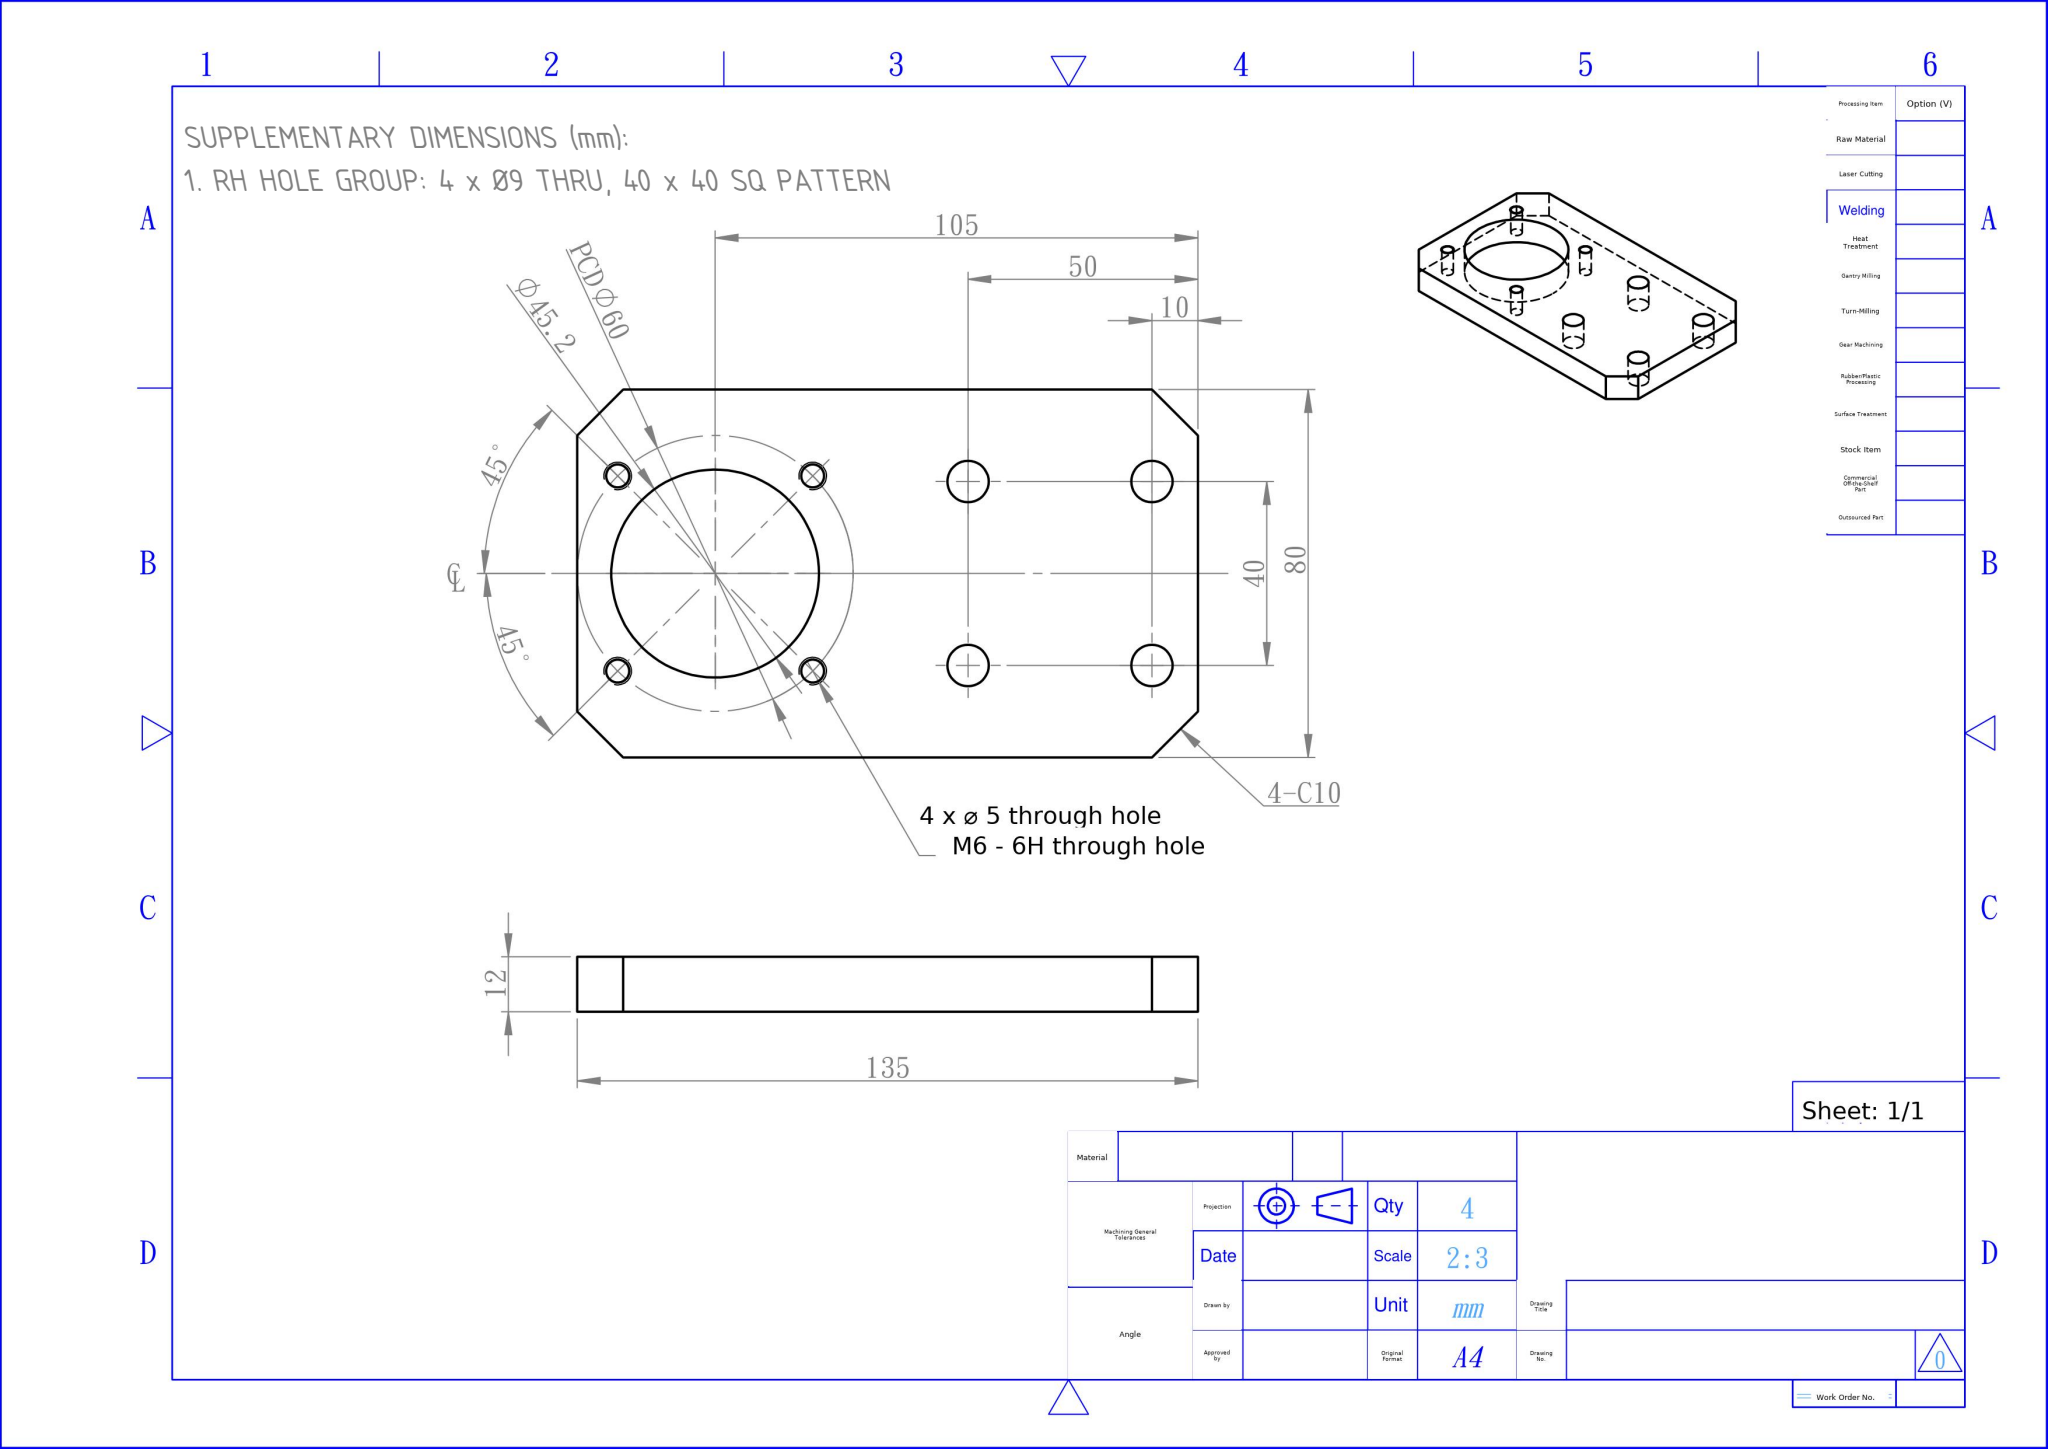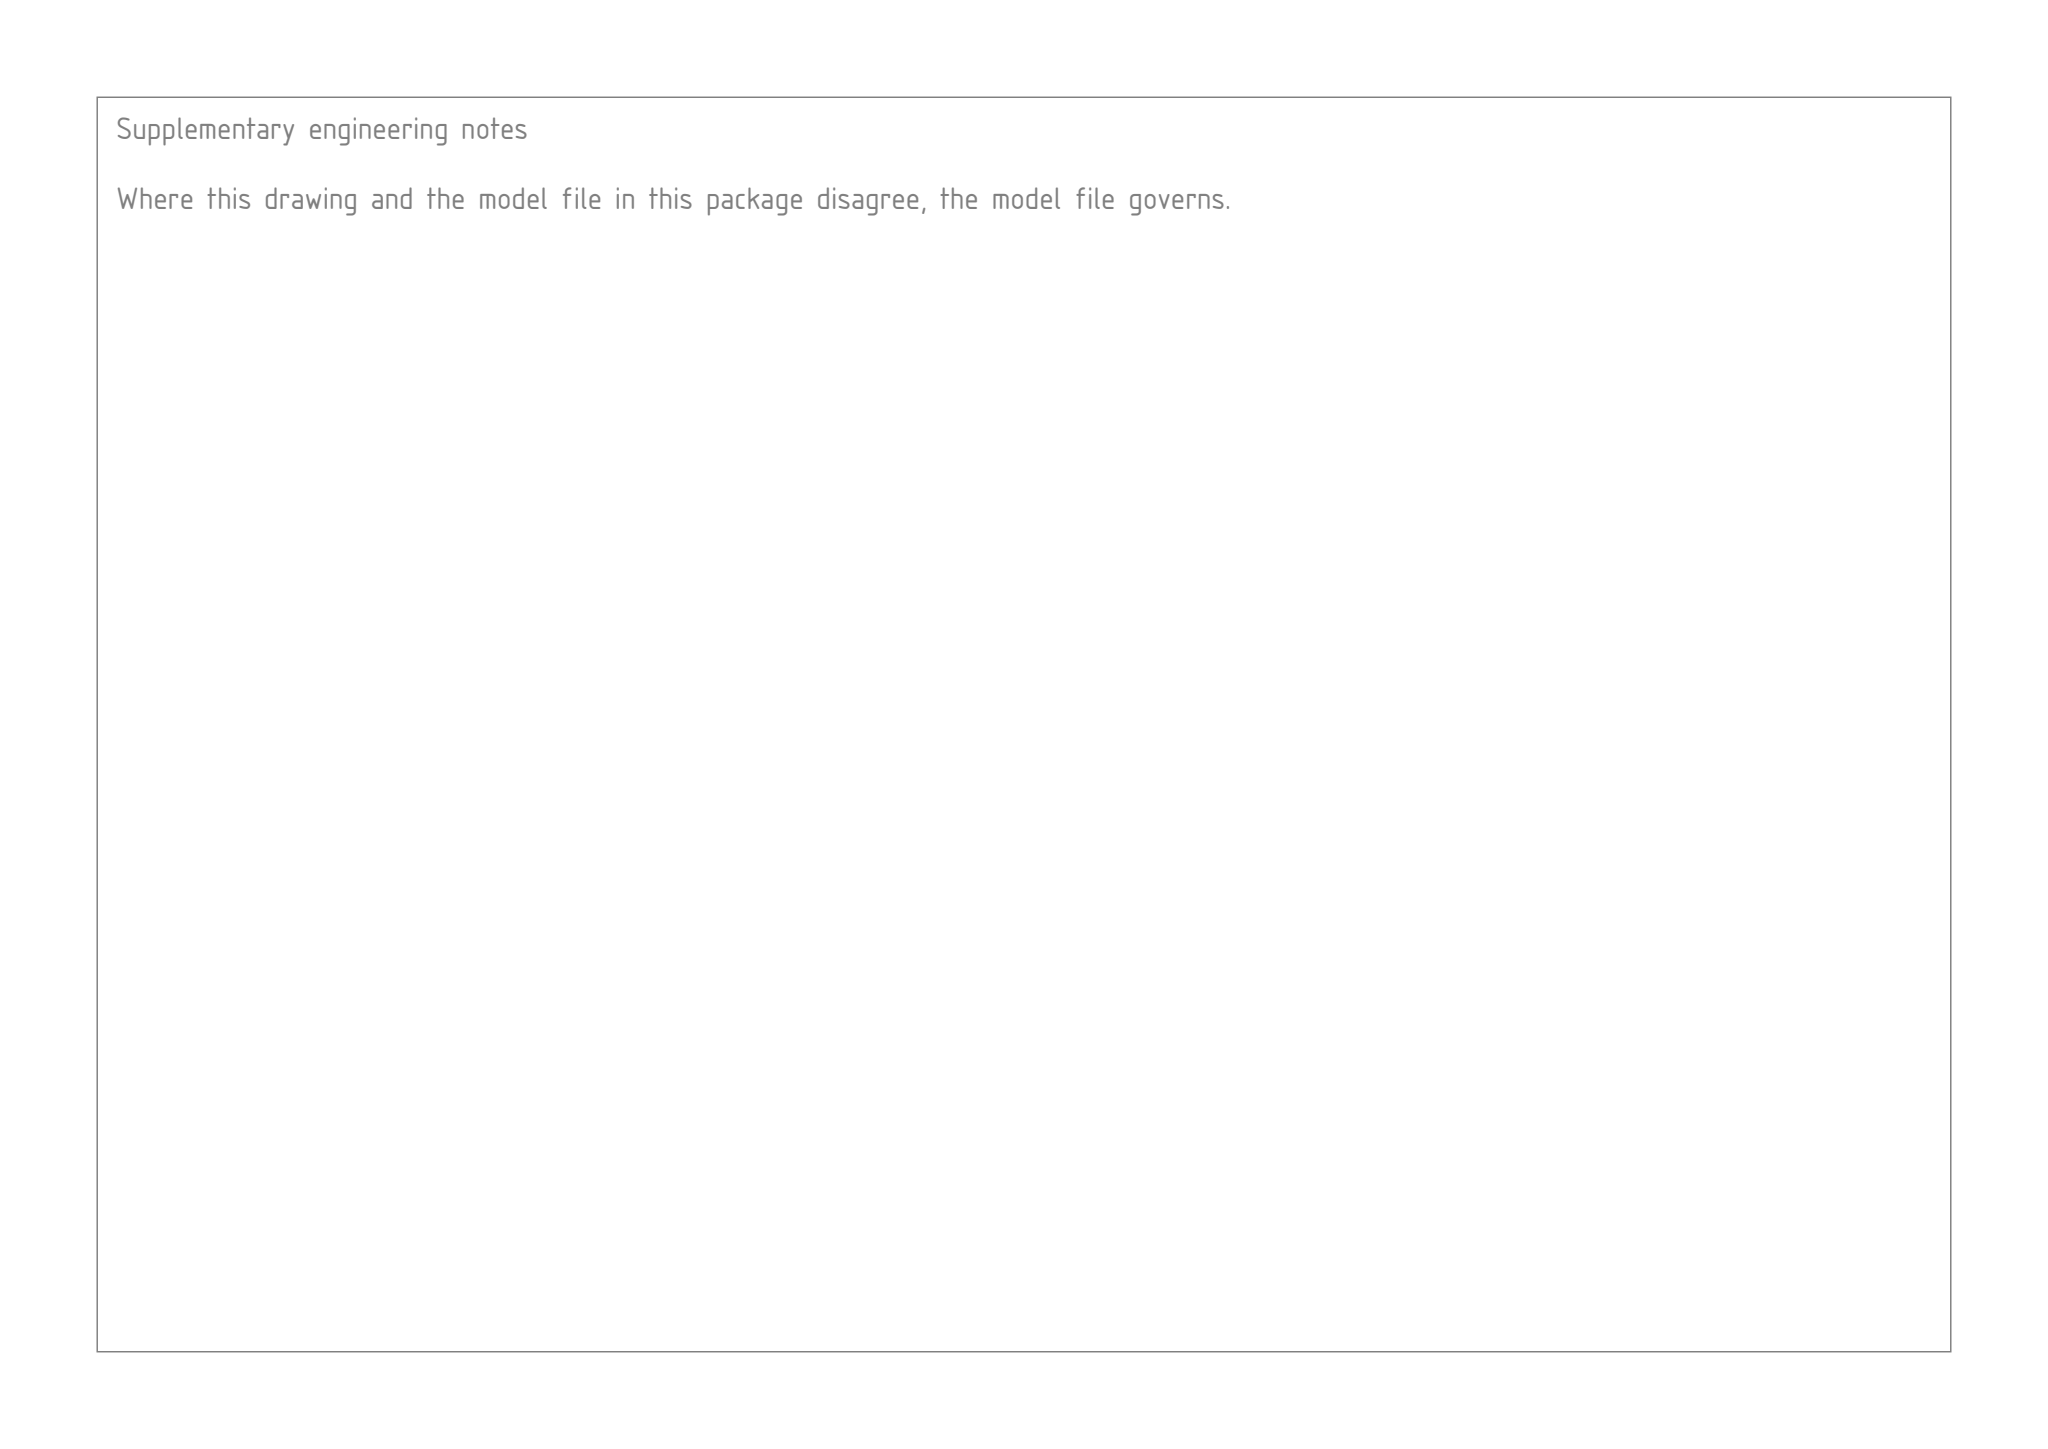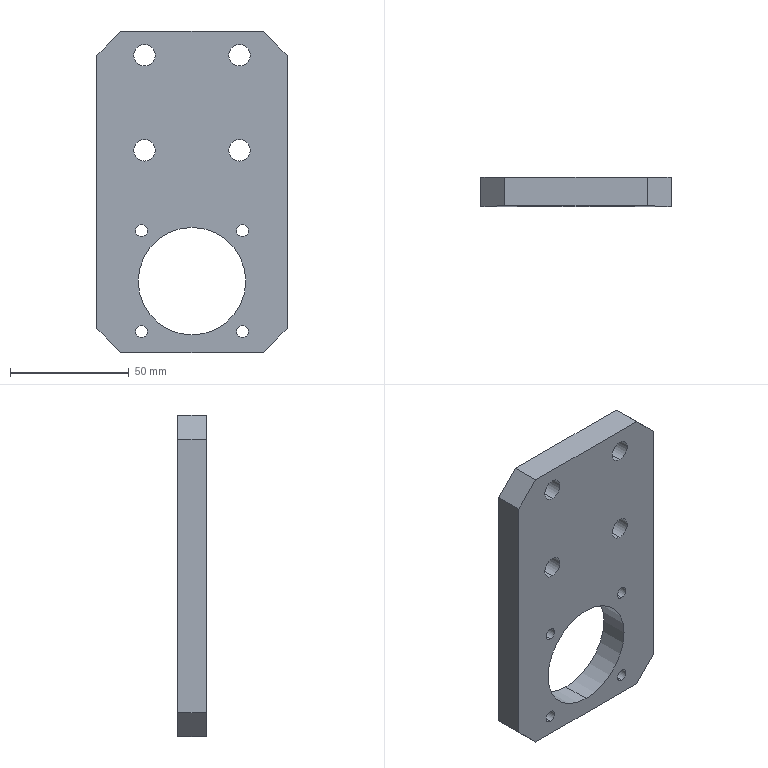Part | SolidWorks | mm | 1 solid | 28 faces | box 80 x 12 x 135 mm | volume 103949 mm3 | cylinder 18 | plane 10 | commonest cylinder face diameters 5 x8 9 x8 45.2 x2
build123d program:
from build123d import *

# Parameters (mm, degrees)
SKETCH1_W                = 80
SKETCH1_H                = 135
BOSS_EXTRUDE1_DEPTH      = 12
F_9_0_9_DIAMETER_HOLE1_D = 9
SKETCH4_R                = 22.6
CUT_EXTRUDE1_DEPTH       = 80.374
M6_TAPPED_HOLE1_D        = 5
CHAMFER1_SIZE            = 10


with BuildPart() as part:
    # Sketch1 → Boss-Extrude1 (new body)
    with BuildSketch(Plane(origin=(0, 0, 0), x_dir=(1, 0, 0), z_dir=(0, 1, 0))):
        Rectangle(SKETCH1_W, SKETCH1_H)
    extrude(amount=BOSS_EXTRUDE1_DEPTH)

    # 9.0 _9_ Diameter Hole1 (through all)
    with Locations(Plane(origin=(0, 12, 0), x_dir=(1, 0, 0), z_dir=(0, 1, 0))):
        with Locations((20, -57.5), (-20, -57.5), (-20, -17.5), (20, -17.5)):
            Hole(F_9_0_9_DIAMETER_HOLE1_D / 2)

    # Sketch4 → Cut-Extrude1 (cut, through all)
    with BuildSketch(Plane(origin=(0, 12, 0), x_dir=(1, 0, 0), z_dir=(0, 1, 0))):
        with Locations(Location((0, 37.5, 0), (0, 0, 270))):
            Circle(SKETCH4_R)
    extrude(amount=-CUT_EXTRUDE1_DEPTH, mode=Mode.SUBTRACT)

    # M6 Tapped Hole1 (through all)
    with Locations(Plane(origin=(0, 12, 0), x_dir=(1, 0, 0), z_dir=(0, 1, 0))):
        with Locations((-21.213, 58.713), (21.213, 58.713), (21.213, 16.287), (-21.213, 16.287)):
            Hole(M6_TAPPED_HOLE1_D / 2)

    # Chamfer1
    chamfer1_edges = [part.edges().sort_by_distance(p)[0] for p in [
        (-40, 6, -67.5),
        (40, 6, -67.5),
        (40, 6, 67.5),
        (-40, 6, 67.5),
    ]]
    chamfer(chamfer1_edges, length=CHAMFER1_SIZE)


solid = part.part